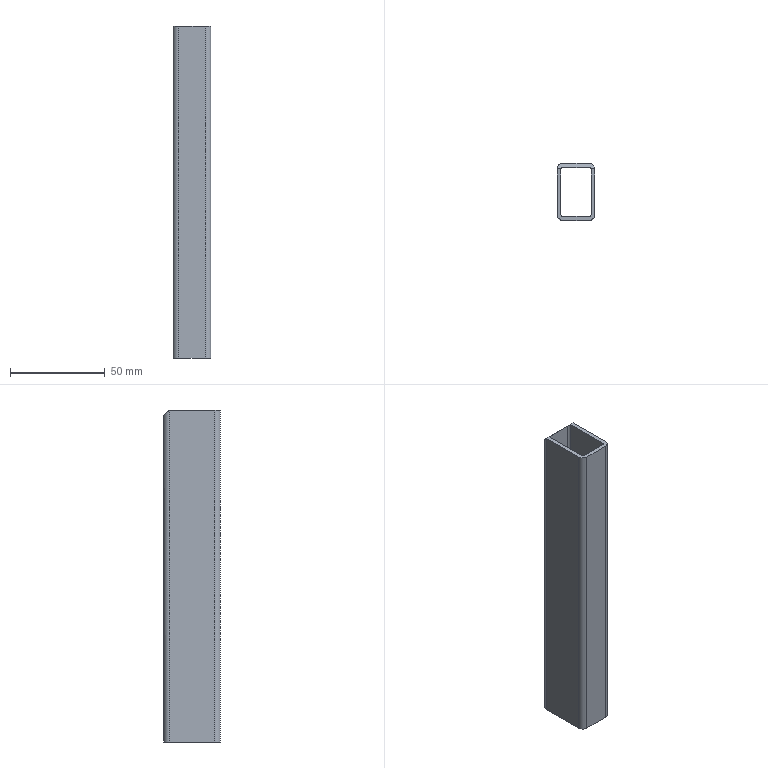Component | SolidWorks | A30x20x2RectangularColdBentHollowSectionSteel175mm-1 | 1 solid | 19 faces | box 20 x 30 x 175 mm | volume 30925 mm3 | plane 11 | cylinder 8 | commonest cylinder face diameters 6 x4 2 x4
build123d program:
from build123d import *

# Parameters (mm, degrees)
BOSS_EXTRUDE1_DEPTH     = 175
CUT_EXTRUDE1_DEPTH      = 176.926
CUT_EXTRUDE1_DEPTH_BACK = 176.926


with BuildPart() as part:
    # Sketch1_2 → Boss-Extrude1 (new body)
    with BuildSketch(Plane(origin=(0, 0, 0), x_dir=(0, 0, -1), z_dir=(1, 0, 0))):
        with BuildLine():
            Line((-6.263, 13), (6.263, 13))
            Line((6.263, 13), (7.561, 14.947))
            ThreePointArc((7.561, 14.947), (7.282, 14.987), (7, 15))
            Line((7, 15), (-7, 15))
            ThreePointArc((-7, 15), (-7.282, 14.987), (-7.561, 14.947))
            Line((-7.561, 14.947), (-6.263, 13))
        make_face()
        with BuildLine():
            Line((-10, -11.394), (-8, -8.394))
            Line((-8, -8.394), (-8, 12))
            ThreePointArc((-8, 12), (-7.707, 12.707), (-7, 13))
            Line((-7, 13), (-6.263, 13))
            Line((-6.263, 13), (-7.561, 14.947))
            ThreePointArc((-7.561, 14.947), (-9.311, 13.913), (-10, 12))
            Line((-10, 12), (-10, -11.394))
        make_face()
        with BuildLine():
            Line((8, 12), (8, -8.394))
            Line((8, -8.394), (10, -11.394))
            Line((10, -11.394), (10, 12))
            ThreePointArc((10, 12), (9.311, 13.913), (7.561, 14.947))
            Line((7.561, 14.947), (6.263, 13))
            Line((6.263, 13), (7, 13))
            ThreePointArc((7, 13), (7.707, 12.707), (8, 12))
        make_face()
        with BuildLine():
            Line((7, -13), (-7, -13))
            ThreePointArc((-7, -13), (-7.707, -12.707), (-8, -12))
            Line((-8, -12), (-8, -8.394))
            Line((-8, -8.394), (-10, -11.394))
            Line((-10, -11.394), (-10, -12))
            ThreePointArc((-10, -12), (-9.121, -14.121), (-7, -15))
            Line((-7, -15), (7, -15))
            ThreePointArc((7, -15), (9.121, -14.121), (10, -12))
            Line((10, -12), (10, -11.394))
            Line((10, -11.394), (8, -8.394))
            Line((8, -8.394), (8, -12))
            ThreePointArc((8, -12), (7.707, -12.707), (7, -13))
        make_face()
    extrude(amount=BOSS_EXTRUDE1_DEPTH)

    # Sketch1 → Cut-Extrude1 (cut, two sides: drawn at the far end of the back side and taken through both)
    with BuildSketch(Plane.XY.offset(-CUT_EXTRUDE1_DEPTH_BACK)):
        Polygon((-1, 11), (-1, 16), (4, 16), align=None)
    extrude(amount=CUT_EXTRUDE1_DEPTH + CUT_EXTRUDE1_DEPTH_BACK, mode=Mode.SUBTRACT)


solid = part.part

# Placed as in the assembly
solid = solid.moved(Location((76.629, 35.1, 413), (0, 90, 0)))
STEP:
#1=COLOUR_RGB('',0.7922,0.8196,0.9333);
#2=FILL_AREA_STYLE_COLOUR('',#1);
#3=FILL_AREA_STYLE('',(#2));
#4=SURFACE_STYLE_FILL_AREA(#3);
#5=SURFACE_SIDE_STYLE('',(#4));
#6=SURFACE_STYLE_USAGE(.BOTH.,#5);
#7=PRESENTATION_STYLE_ASSIGNMENT((#6));
#8=CARTESIAN_POINT('',(3.411,1.854,16.26));
#9=VERTEX_POINT('',#8);
#10=CARTESIAN_POINT('',(3.292,1.972,16.142));
#11=VERTEX_POINT('',#10);
#12=CARTESIAN_POINT('',(3.411,1.854,16.26));
#13=CARTESIAN_POINT('',(3.411,1.924,16.191));
#14=CARTESIAN_POINT('',(3.362,1.972,16.142));
#15=CARTESIAN_POINT('',(3.292,1.972,16.142));
#16=(BOUNDED_CURVE()B_SPLINE_CURVE(3,(#12,#13,#14,#15),.UNSPECIFIED.,.F.,.T.)B_SPLINE_CURVE_WITH_KNOTS((4,4),(1.571,3.142),.UNSPECIFIED.)CURVE()GEOMETRIC_REPRESENTATION_ITEM()RATIONAL_B_SPLINE_CURVE((1.,0.8047,0.8047,1.))REPRESENTATION_ITEM(''));
#17=EDGE_CURVE('',#9,#11,#16,.T.);
#18=ORIENTED_EDGE('',*,*,#17,.F.);
#19=CARTESIAN_POINT('',(3.411,1.854,9.37));
#20=VERTEX_POINT('',#19);
#21=CARTESIAN_POINT('',(3.411,1.854,9.37));
#22=DIRECTION('',(-0.,-0.,1.));
#23=VECTOR('',#22,39.37);
#24=LINE('',#21,#23);
#25=EDGE_CURVE('',#20,#9,#24,.T.);
#26=ORIENTED_EDGE('',*,*,#25,.F.);
#27=CARTESIAN_POINT('',(3.292,1.972,9.37));
#28=VERTEX_POINT('',#27);
#29=CARTESIAN_POINT('',(3.292,1.854,9.37));
#30=DIRECTION('',(-0.,-0.,1.));
#31=DIRECTION('',(-1.,0.,0.));
#32=AXIS2_PLACEMENT_3D('',#29,#30,#31);
#33=CIRCLE('',#32,0.1181);
#34=EDGE_CURVE('',#20,#28,#33,.T.);
#35=ORIENTED_EDGE('',*,*,#34,.T.);
#36=CARTESIAN_POINT('',(3.292,1.972,9.37));
#37=DIRECTION('',(-0.,-0.,1.));
#38=VECTOR('',#37,39.37);
#39=LINE('',#36,#38);
#40=EDGE_CURVE('',#28,#11,#39,.T.);
#41=ORIENTED_EDGE('',*,*,#40,.T.);
#42=EDGE_LOOP('',(#18,#26,#35,#41));
#43=FACE_OUTER_BOUND('',#42,.T.);
#44=CARTESIAN_POINT('',(3.292,1.854,9.37));
#45=DIRECTION('',(-0.,-0.,1.));
#46=DIRECTION('',(1.,0.,0.));
#47=AXIS2_PLACEMENT_3D('',#44,#45,#46);
#48=CYLINDRICAL_SURFACE('',#47,0.1181);
#49=ADVANCED_FACE('',(#43),#48,.T.);
#50=CARTESIAN_POINT('',(3.411,0.9094,16.26));
#51=VERTEX_POINT('',#50);
#52=CARTESIAN_POINT('',(3.411,1.382,16.26));
#53=DIRECTION('',(0.,1.,0.));
#54=VECTOR('',#53,39.37);
#55=LINE('',#52,#54);
#56=EDGE_CURVE('',#51,#9,#55,.T.);
#57=ORIENTED_EDGE('',*,*,#56,.F.);
#58=CARTESIAN_POINT('',(3.411,0.9094,9.37));
#59=VERTEX_POINT('',#58);
#60=CARTESIAN_POINT('',(3.411,0.9094,9.37));
#61=DIRECTION('',(-0.,-0.,1.));
#62=VECTOR('',#61,39.37);
#63=LINE('',#60,#62);
#64=EDGE_CURVE('',#59,#51,#63,.T.);
#65=ORIENTED_EDGE('',*,*,#64,.F.);
#66=CARTESIAN_POINT('',(3.411,1.382,9.37));
#67=DIRECTION('',(0.,1.,0.));
#68=VECTOR('',#67,39.37);
#69=LINE('',#66,#68);
#70=EDGE_CURVE('',#59,#20,#69,.T.);
#71=ORIENTED_EDGE('',*,*,#70,.T.);
#72=ORIENTED_EDGE('',*,*,#25,.T.);
#73=EDGE_LOOP('',(#57,#65,#71,#72));
#74=FACE_OUTER_BOUND('',#73,.T.);
#75=CARTESIAN_POINT('',(3.411,1.382,9.37));
#76=DIRECTION('',(1.,-0.,0.));
#77=DIRECTION('',(0.,0.,-1.));
#78=AXIS2_PLACEMENT_3D('',#75,#76,#77);
#79=PLANE('',#78);
#80=ADVANCED_FACE('',(#74),#79,.T.);
#81=CARTESIAN_POINT('',(3.292,0.7913,16.26));
#82=VERTEX_POINT('',#81);
#83=CARTESIAN_POINT('',(3.292,0.9094,16.26));
#84=DIRECTION('',(-0.,-0.,1.));
#85=DIRECTION('',(-1.,0.,0.));
#86=AXIS2_PLACEMENT_3D('',#83,#84,#85);
#87=CIRCLE('',#86,0.1181);
#88=EDGE_CURVE('',#82,#51,#87,.T.);
#89=ORIENTED_EDGE('',*,*,#88,.F.);
#90=CARTESIAN_POINT('',(3.292,0.7913,9.37));
#91=VERTEX_POINT('',#90);
#92=CARTESIAN_POINT('',(3.292,0.7913,9.37));
#93=DIRECTION('',(-0.,-0.,1.));
#94=VECTOR('',#93,39.37);
#95=LINE('',#92,#94);
#96=EDGE_CURVE('',#91,#82,#95,.T.);
#97=ORIENTED_EDGE('',*,*,#96,.F.);
#98=CARTESIAN_POINT('',(3.292,0.9094,9.37));
#99=DIRECTION('',(-0.,-0.,1.));
#100=DIRECTION('',(-1.,0.,0.));
#101=AXIS2_PLACEMENT_3D('',#98,#99,#100);
#102=CIRCLE('',#101,0.1181);
#103=EDGE_CURVE('',#91,#59,#102,.T.);
#104=ORIENTED_EDGE('',*,*,#103,.T.);
#105=ORIENTED_EDGE('',*,*,#64,.T.);
#106=EDGE_LOOP('',(#89,#97,#104,#105));
#107=FACE_OUTER_BOUND('',#106,.T.);
#108=CARTESIAN_POINT('',(3.292,0.9094,9.37));
#109=DIRECTION('',(-0.,-0.,1.));
#110=DIRECTION('',(1.,0.,0.));
#111=AXIS2_PLACEMENT_3D('',#108,#109,#110);
#112=CYLINDRICAL_SURFACE('',#111,0.1181);
#113=ADVANCED_FACE('',(#107),#112,.T.);
#114=CARTESIAN_POINT('',(2.741,0.7913,16.26));
#115=VERTEX_POINT('',#114);
#116=CARTESIAN_POINT('',(3.017,0.7913,16.26));
#117=DIRECTION('',(-1.,0.,-0.));
#118=VECTOR('',#117,39.37);
#119=LINE('',#116,#118);
#120=EDGE_CURVE('',#82,#115,#119,.T.);
#121=ORIENTED_EDGE('',*,*,#120,.T.);
#122=CARTESIAN_POINT('',(2.741,0.7913,9.37));
#123=VERTEX_POINT('',#122);
#124=CARTESIAN_POINT('',(2.741,0.7913,9.37));
#125=DIRECTION('',(-0.,-0.,1.));
#126=VECTOR('',#125,39.37);
#127=LINE('',#124,#126);
#128=EDGE_CURVE('',#123,#115,#127,.T.);
#129=ORIENTED_EDGE('',*,*,#128,.F.);
#130=CARTESIAN_POINT('',(3.017,0.7913,9.37));
#131=DIRECTION('',(-1.,0.,-0.));
#132=VECTOR('',#131,39.37);
#133=LINE('',#130,#132);
#134=EDGE_CURVE('',#91,#123,#133,.T.);
#135=ORIENTED_EDGE('',*,*,#134,.F.);
#136=ORIENTED_EDGE('',*,*,#96,.T.);
#137=EDGE_LOOP('',(#121,#129,#135,#136));
#138=FACE_OUTER_BOUND('',#137,.T.);
#139=CARTESIAN_POINT('',(3.017,0.7913,9.37));
#140=DIRECTION('',(0.,1.,0.));
#141=DIRECTION('',(1.,-0.,0.));
#142=AXIS2_PLACEMENT_3D('',#139,#140,#141);
#143=PLANE('',#142);
#144=ADVANCED_FACE('',(#138),#143,.F.);
#145=CARTESIAN_POINT('',(2.623,0.9094,16.26));
#146=VERTEX_POINT('',#145);
#147=CARTESIAN_POINT('',(2.741,0.9094,16.26));
#148=DIRECTION('',(0.,0.,-1.));
#149=DIRECTION('',(-1.,0.,0.));
#150=AXIS2_PLACEMENT_3D('',#147,#148,#149);
#151=CIRCLE('',#150,0.1181);
#152=EDGE_CURVE('',#115,#146,#151,.T.);
#153=ORIENTED_EDGE('',*,*,#152,.T.);
#154=CARTESIAN_POINT('',(2.623,0.9094,9.37));
#155=VERTEX_POINT('',#154);
#156=CARTESIAN_POINT('',(2.623,0.9094,9.37));
#157=DIRECTION('',(-0.,-0.,1.));
#158=VECTOR('',#157,39.37);
#159=LINE('',#156,#158);
#160=EDGE_CURVE('',#155,#146,#159,.T.);
#161=ORIENTED_EDGE('',*,*,#160,.F.);
#162=CARTESIAN_POINT('',(2.741,0.9094,9.37));
#163=DIRECTION('',(0.,0.,-1.));
#164=DIRECTION('',(-1.,0.,0.));
#165=AXIS2_PLACEMENT_3D('',#162,#163,#164);
#166=CIRCLE('',#165,0.1181);
#167=EDGE_CURVE('',#123,#155,#166,.T.);
#168=ORIENTED_EDGE('',*,*,#167,.F.);
#169=ORIENTED_EDGE('',*,*,#128,.T.);
#170=EDGE_LOOP('',(#153,#161,#168,#169));
#171=FACE_OUTER_BOUND('',#170,.T.);
#172=CARTESIAN_POINT('',(2.741,0.9094,9.37));
#173=DIRECTION('',(-0.,-0.,1.));
#174=DIRECTION('',(1.,0.,0.));
#175=AXIS2_PLACEMENT_3D('',#172,#173,#174);
#176=CYLINDRICAL_SURFACE('',#175,0.1181);
#177=ADVANCED_FACE('',(#171),#176,.T.);
#178=CARTESIAN_POINT('',(2.623,1.854,16.26));
#179=VERTEX_POINT('',#178);
#180=CARTESIAN_POINT('',(2.623,1.382,16.26));
#181=DIRECTION('',(0.,1.,0.));
#182=VECTOR('',#181,39.37);
#183=LINE('',#180,#182);
#184=EDGE_CURVE('',#146,#179,#183,.T.);
#185=ORIENTED_EDGE('',*,*,#184,.T.);
#186=CARTESIAN_POINT('',(2.623,1.854,9.37));
#187=VERTEX_POINT('',#186);
#188=CARTESIAN_POINT('',(2.623,1.854,9.37));
#189=DIRECTION('',(-0.,-0.,1.));
#190=VECTOR('',#189,39.37);
#191=LINE('',#188,#190);
#192=EDGE_CURVE('',#187,#179,#191,.T.);
#193=ORIENTED_EDGE('',*,*,#192,.F.);
#194=CARTESIAN_POINT('',(2.623,1.382,9.37));
#195=DIRECTION('',(0.,1.,0.));
#196=VECTOR('',#195,39.37);
#197=LINE('',#194,#196);
#198=EDGE_CURVE('',#155,#187,#197,.T.);
#199=ORIENTED_EDGE('',*,*,#198,.F.);
#200=ORIENTED_EDGE('',*,*,#160,.T.);
#201=EDGE_LOOP('',(#185,#193,#199,#200));
#202=FACE_OUTER_BOUND('',#201,.T.);
#203=CARTESIAN_POINT('',(2.623,1.382,9.37));
#204=DIRECTION('',(1.,-0.,0.));
#205=DIRECTION('',(0.,0.,-1.));
#206=AXIS2_PLACEMENT_3D('',#203,#204,#205);
#207=PLANE('',#206);
#208=ADVANCED_FACE('',(#202),#207,.F.);
#209=CARTESIAN_POINT('',(2.741,1.972,16.142));
#210=VERTEX_POINT('',#209);
#211=CARTESIAN_POINT('',(2.741,1.972,16.142));
#212=CARTESIAN_POINT('',(2.672,1.972,16.142));
#213=CARTESIAN_POINT('',(2.623,1.924,16.191));
#214=CARTESIAN_POINT('',(2.623,1.854,16.26));
#215=(BOUNDED_CURVE()B_SPLINE_CURVE(3,(#211,#212,#213,#214),.UNSPECIFIED.,.F.,.T.)B_SPLINE_CURVE_WITH_KNOTS((4,4),(3.142,4.712),.UNSPECIFIED.)CURVE()GEOMETRIC_REPRESENTATION_ITEM()RATIONAL_B_SPLINE_CURVE((1.,0.8047,0.8047,1.))REPRESENTATION_ITEM(''));
#216=EDGE_CURVE('',#210,#179,#215,.T.);
#217=ORIENTED_EDGE('',*,*,#216,.F.);
#218=CARTESIAN_POINT('',(2.741,1.972,9.37));
#219=VERTEX_POINT('',#218);
#220=CARTESIAN_POINT('',(2.741,1.972,9.37));
#221=DIRECTION('',(-0.,-0.,1.));
#222=VECTOR('',#221,39.37);
#223=LINE('',#220,#222);
#224=EDGE_CURVE('',#219,#210,#223,.T.);
#225=ORIENTED_EDGE('',*,*,#224,.F.);
#226=CARTESIAN_POINT('',(2.741,1.854,9.37));
#227=DIRECTION('',(-0.,-0.,1.));
#228=DIRECTION('',(-1.,0.,0.));
#229=AXIS2_PLACEMENT_3D('',#226,#227,#228);
#230=CIRCLE('',#229,0.1181);
#231=EDGE_CURVE('',#219,#187,#230,.T.);
#232=ORIENTED_EDGE('',*,*,#231,.T.);
#233=ORIENTED_EDGE('',*,*,#192,.T.);
#234=EDGE_LOOP('',(#217,#225,#232,#233));
#235=FACE_OUTER_BOUND('',#234,.T.);
#236=CARTESIAN_POINT('',(2.741,1.854,9.37));
#237=DIRECTION('',(-0.,-0.,1.));
#238=DIRECTION('',(1.,0.,0.));
#239=AXIS2_PLACEMENT_3D('',#236,#237,#238);
#240=CYLINDRICAL_SURFACE('',#239,0.1181);
#241=ADVANCED_FACE('',(#235),#240,.T.);
#242=CARTESIAN_POINT('',(3.292,0.8701,16.26));
#243=VERTEX_POINT('',#242);
#244=CARTESIAN_POINT('',(3.332,0.9094,16.26));
#245=VERTEX_POINT('',#244);
#246=CARTESIAN_POINT('',(3.292,0.9094,16.26));
#247=DIRECTION('',(-0.,-0.,1.));
#248=DIRECTION('',(-1.,0.,0.));
#249=AXIS2_PLACEMENT_3D('',#246,#247,#248);
#250=CIRCLE('',#249,0.03937);
#251=EDGE_CURVE('',#243,#245,#250,.T.);
#252=ORIENTED_EDGE('',*,*,#251,.T.);
#253=CARTESIAN_POINT('',(3.332,0.9094,9.37));
#254=VERTEX_POINT('',#253);
#255=CARTESIAN_POINT('',(3.332,0.9094,9.37));
#256=DIRECTION('',(-0.,-0.,1.));
#257=VECTOR('',#256,39.37);
#258=LINE('',#255,#257);
#259=EDGE_CURVE('',#254,#245,#258,.T.);
#260=ORIENTED_EDGE('',*,*,#259,.F.);
#261=CARTESIAN_POINT('',(3.292,0.8701,9.37));
#262=VERTEX_POINT('',#261);
#263=CARTESIAN_POINT('',(3.292,0.9094,9.37));
#264=DIRECTION('',(-0.,-0.,1.));
#265=DIRECTION('',(-1.,0.,0.));
#266=AXIS2_PLACEMENT_3D('',#263,#264,#265);
#267=CIRCLE('',#266,0.03937);
#268=EDGE_CURVE('',#262,#254,#267,.T.);
#269=ORIENTED_EDGE('',*,*,#268,.F.);
#270=CARTESIAN_POINT('',(3.292,0.8701,9.37));
#271=DIRECTION('',(-0.,-0.,1.));
#272=VECTOR('',#271,39.37);
#273=LINE('',#270,#272);
#274=EDGE_CURVE('',#262,#243,#273,.T.);
#275=ORIENTED_EDGE('',*,*,#274,.T.);
#276=EDGE_LOOP('',(#252,#260,#269,#275));
#277=FACE_OUTER_BOUND('',#276,.T.);
#278=CARTESIAN_POINT('',(3.292,0.9094,9.37));
#279=DIRECTION('',(-0.,-0.,1.));
#280=DIRECTION('',(1.,0.,0.));
#281=AXIS2_PLACEMENT_3D('',#278,#279,#280);
#282=CYLINDRICAL_SURFACE('',#281,0.03937);
#283=ADVANCED_FACE('',(#277),#282,.F.);
#284=CARTESIAN_POINT('',(3.332,1.854,16.26));
#285=VERTEX_POINT('',#284);
#286=CARTESIAN_POINT('',(3.332,1.382,16.26));
#287=DIRECTION('',(0.,1.,0.));
#288=VECTOR('',#287,39.37);
#289=LINE('',#286,#288);
#290=EDGE_CURVE('',#245,#285,#289,.T.);
#291=ORIENTED_EDGE('',*,*,#290,.T.);
#292=CARTESIAN_POINT('',(3.332,1.854,9.37));
#293=VERTEX_POINT('',#292);
#294=CARTESIAN_POINT('',(3.332,1.854,9.37));
#295=DIRECTION('',(-0.,-0.,1.));
#296=VECTOR('',#295,39.37);
#297=LINE('',#294,#296);
#298=EDGE_CURVE('',#293,#285,#297,.T.);
#299=ORIENTED_EDGE('',*,*,#298,.F.);
#300=CARTESIAN_POINT('',(3.332,1.382,9.37));
#301=DIRECTION('',(0.,1.,0.));
#302=VECTOR('',#301,39.37);
#303=LINE('',#300,#302);
#304=EDGE_CURVE('',#254,#293,#303,.T.);
#305=ORIENTED_EDGE('',*,*,#304,.F.);
#306=ORIENTED_EDGE('',*,*,#259,.T.);
#307=EDGE_LOOP('',(#291,#299,#305,#306));
#308=FACE_OUTER_BOUND('',#307,.T.);
#309=CARTESIAN_POINT('',(3.332,1.382,9.37));
#310=DIRECTION('',(1.,-0.,0.));
#311=DIRECTION('',(0.,0.,-1.));
#312=AXIS2_PLACEMENT_3D('',#309,#310,#311);
#313=PLANE('',#312);
#314=ADVANCED_FACE('',(#308),#313,.F.);
#315=ORIENTED_EDGE('',*,*,#298,.T.);
#316=CARTESIAN_POINT('',(3.292,1.894,16.22));
#317=VERTEX_POINT('',#316);
#318=CARTESIAN_POINT('',(3.332,1.854,16.26));
#319=CARTESIAN_POINT('',(3.332,1.877,16.237));
#320=CARTESIAN_POINT('',(3.316,1.894,16.22));
#321=CARTESIAN_POINT('',(3.292,1.894,16.22));
#322=(BOUNDED_CURVE()B_SPLINE_CURVE(3,(#318,#319,#320,#321),.UNSPECIFIED.,.F.,.T.)B_SPLINE_CURVE_WITH_KNOTS((4,4),(1.571,3.142),.UNSPECIFIED.)CURVE()GEOMETRIC_REPRESENTATION_ITEM()RATIONAL_B_SPLINE_CURVE((1.,0.8047,0.8047,1.))REPRESENTATION_ITEM(''));
#323=EDGE_CURVE('',#285,#317,#322,.T.);
#324=ORIENTED_EDGE('',*,*,#323,.T.);
#325=CARTESIAN_POINT('',(3.292,1.894,9.37));
#326=VERTEX_POINT('',#325);
#327=CARTESIAN_POINT('',(3.292,1.894,9.37));
#328=DIRECTION('',(-0.,-0.,1.));
#329=VECTOR('',#328,39.37);
#330=LINE('',#327,#329);
#331=EDGE_CURVE('',#326,#317,#330,.T.);
#332=ORIENTED_EDGE('',*,*,#331,.F.);
#333=CARTESIAN_POINT('',(3.292,1.854,9.37));
#334=DIRECTION('',(-0.,-0.,1.));
#335=DIRECTION('',(-1.,0.,0.));
#336=AXIS2_PLACEMENT_3D('',#333,#334,#335);
#337=CIRCLE('',#336,0.03937);
#338=EDGE_CURVE('',#293,#326,#337,.T.);
#339=ORIENTED_EDGE('',*,*,#338,.F.);
#340=EDGE_LOOP('',(#315,#324,#332,#339));
#341=FACE_OUTER_BOUND('',#340,.T.);
#342=CARTESIAN_POINT('',(3.292,1.854,9.37));
#343=DIRECTION('',(-0.,-0.,1.));
#344=DIRECTION('',(1.,0.,0.));
#345=AXIS2_PLACEMENT_3D('',#342,#343,#344);
#346=CYLINDRICAL_SURFACE('',#345,0.03937);
#347=ADVANCED_FACE('',(#341),#346,.F.);
#348=ORIENTED_EDGE('',*,*,#331,.T.);
#349=CARTESIAN_POINT('',(2.741,1.894,16.22));
#350=VERTEX_POINT('',#349);
#351=CARTESIAN_POINT('',(3.017,1.894,16.22));
#352=DIRECTION('',(-1.,0.,-0.));
#353=VECTOR('',#352,39.37);
#354=LINE('',#351,#353);
#355=EDGE_CURVE('',#317,#350,#354,.T.);
#356=ORIENTED_EDGE('',*,*,#355,.T.);
#357=CARTESIAN_POINT('',(2.741,1.894,9.37));
#358=VERTEX_POINT('',#357);
#359=CARTESIAN_POINT('',(2.741,1.894,9.37));
#360=DIRECTION('',(-0.,-0.,1.));
#361=VECTOR('',#360,39.37);
#362=LINE('',#359,#361);
#363=EDGE_CURVE('',#358,#350,#362,.T.);
#364=ORIENTED_EDGE('',*,*,#363,.F.);
#365=CARTESIAN_POINT('',(3.017,1.894,9.37));
#366=DIRECTION('',(-1.,0.,-0.));
#367=VECTOR('',#366,39.37);
#368=LINE('',#365,#367);
#369=EDGE_CURVE('',#326,#358,#368,.T.);
#370=ORIENTED_EDGE('',*,*,#369,.F.);
#371=EDGE_LOOP('',(#348,#356,#364,#370));
#372=FACE_OUTER_BOUND('',#371,.T.);
#373=CARTESIAN_POINT('',(3.017,1.894,9.37));
#374=DIRECTION('',(0.,1.,0.));
#375=DIRECTION('',(1.,-0.,0.));
#376=AXIS2_PLACEMENT_3D('',#373,#374,#375);
#377=PLANE('',#376);
#378=ADVANCED_FACE('',(#372),#377,.F.);
#379=ORIENTED_EDGE('',*,*,#363,.T.);
#380=CARTESIAN_POINT('',(2.702,1.854,16.26));
#381=VERTEX_POINT('',#380);
#382=CARTESIAN_POINT('',(2.741,1.894,16.22));
#383=CARTESIAN_POINT('',(2.718,1.894,16.22));
#384=CARTESIAN_POINT('',(2.702,1.877,16.237));
#385=CARTESIAN_POINT('',(2.702,1.854,16.26));
#386=(BOUNDED_CURVE()B_SPLINE_CURVE(3,(#382,#383,#384,#385),.UNSPECIFIED.,.F.,.T.)B_SPLINE_CURVE_WITH_KNOTS((4,4),(3.142,4.712),.UNSPECIFIED.)CURVE()GEOMETRIC_REPRESENTATION_ITEM()RATIONAL_B_SPLINE_CURVE((1.,0.8047,0.8047,1.))REPRESENTATION_ITEM(''));
#387=EDGE_CURVE('',#350,#381,#386,.T.);
#388=ORIENTED_EDGE('',*,*,#387,.T.);
#389=CARTESIAN_POINT('',(2.702,1.854,9.37));
#390=VERTEX_POINT('',#389);
#391=CARTESIAN_POINT('',(2.702,1.854,9.37));
#392=DIRECTION('',(-0.,-0.,1.));
#393=VECTOR('',#392,39.37);
#394=LINE('',#391,#393);
#395=EDGE_CURVE('',#390,#381,#394,.T.);
#396=ORIENTED_EDGE('',*,*,#395,.F.);
#397=CARTESIAN_POINT('',(2.741,1.854,9.37));
#398=DIRECTION('',(-0.,-0.,1.));
#399=DIRECTION('',(-1.,0.,0.));
#400=AXIS2_PLACEMENT_3D('',#397,#398,#399);
#401=CIRCLE('',#400,0.03937);
#402=EDGE_CURVE('',#358,#390,#401,.T.);
#403=ORIENTED_EDGE('',*,*,#402,.F.);
#404=EDGE_LOOP('',(#379,#388,#396,#403));
#405=FACE_OUTER_BOUND('',#404,.T.);
#406=CARTESIAN_POINT('',(2.741,1.854,9.37));
#407=DIRECTION('',(-0.,-0.,1.));
#408=DIRECTION('',(1.,0.,0.));
#409=AXIS2_PLACEMENT_3D('',#406,#407,#408);
#410=CYLINDRICAL_SURFACE('',#409,0.03937);
#411=ADVANCED_FACE('',(#405),#410,.F.);
#412=CARTESIAN_POINT('',(2.702,0.9094,16.26));
#413=VERTEX_POINT('',#412);
#414=CARTESIAN_POINT('',(2.702,1.382,16.26));
#415=DIRECTION('',(0.,1.,0.));
#416=VECTOR('',#415,39.37);
#417=LINE('',#414,#416);
#418=EDGE_CURVE('',#413,#381,#417,.T.);
#419=ORIENTED_EDGE('',*,*,#418,.F.);
#420=CARTESIAN_POINT('',(2.702,0.9094,9.37));
#421=VERTEX_POINT('',#420);
#422=CARTESIAN_POINT('',(2.702,0.9094,9.37));
#423=DIRECTION('',(-0.,-0.,1.));
#424=VECTOR('',#423,39.37);
#425=LINE('',#422,#424);
#426=EDGE_CURVE('',#421,#413,#425,.T.);
#427=ORIENTED_EDGE('',*,*,#426,.F.);
#428=CARTESIAN_POINT('',(2.702,1.382,9.37));
#429=DIRECTION('',(0.,1.,0.));
#430=VECTOR('',#429,39.37);
#431=LINE('',#428,#430);
#432=EDGE_CURVE('',#421,#390,#431,.T.);
#433=ORIENTED_EDGE('',*,*,#432,.T.);
#434=ORIENTED_EDGE('',*,*,#395,.T.);
#435=EDGE_LOOP('',(#419,#427,#433,#434));
#436=FACE_OUTER_BOUND('',#435,.T.);
#437=CARTESIAN_POINT('',(2.702,1.382,9.37));
#438=DIRECTION('',(1.,-0.,0.));
#439=DIRECTION('',(0.,0.,-1.));
#440=AXIS2_PLACEMENT_3D('',#437,#438,#439);
#441=PLANE('',#440);
#442=ADVANCED_FACE('',(#436),#441,.T.);
#443=CARTESIAN_POINT('',(2.741,0.8701,16.26));
#444=VERTEX_POINT('',#443);
#445=CARTESIAN_POINT('',(2.741,0.9094,16.26));
#446=DIRECTION('',(0.,0.,-1.));
#447=DIRECTION('',(-1.,0.,0.));
#448=AXIS2_PLACEMENT_3D('',#445,#446,#447);
#449=CIRCLE('',#448,0.03937);
#450=EDGE_CURVE('',#444,#413,#449,.T.);
#451=ORIENTED_EDGE('',*,*,#450,.F.);
#452=CARTESIAN_POINT('',(2.741,0.8701,9.37));
#453=VERTEX_POINT('',#452);
#454=CARTESIAN_POINT('',(2.741,0.8701,9.37));
#455=DIRECTION('',(-0.,-0.,1.));
#456=VECTOR('',#455,39.37);
#457=LINE('',#454,#456);
#458=EDGE_CURVE('',#453,#444,#457,.T.);
#459=ORIENTED_EDGE('',*,*,#458,.F.);
#460=CARTESIAN_POINT('',(2.741,0.9094,9.37));
#461=DIRECTION('',(0.,0.,-1.));
#462=DIRECTION('',(-1.,0.,0.));
#463=AXIS2_PLACEMENT_3D('',#460,#461,#462);
#464=CIRCLE('',#463,0.03937);
#465=EDGE_CURVE('',#453,#421,#464,.T.);
#466=ORIENTED_EDGE('',*,*,#465,.T.);
#467=ORIENTED_EDGE('',*,*,#426,.T.);
#468=EDGE_LOOP('',(#451,#459,#466,#467));
#469=FACE_OUTER_BOUND('',#468,.T.);
#470=CARTESIAN_POINT('',(2.741,0.9094,9.37));
#471=DIRECTION('',(-0.,-0.,1.));
#472=DIRECTION('',(1.,0.,0.));
#473=AXIS2_PLACEMENT_3D('',#470,#471,#472);
#474=CYLINDRICAL_SURFACE('',#473,0.03937);
#475=ADVANCED_FACE('',(#469),#474,.F.);
#476=CARTESIAN_POINT('',(3.017,0.8701,16.26));
#477=DIRECTION('',(-1.,0.,-0.));
#478=VECTOR('',#477,39.37);
#479=LINE('',#476,#478);
#480=EDGE_CURVE('',#243,#444,#479,.T.);
#481=ORIENTED_EDGE('',*,*,#480,.F.);
#482=ORIENTED_EDGE('',*,*,#274,.F.);
#483=CARTESIAN_POINT('',(3.017,0.8701,9.37));
#484=DIRECTION('',(-1.,0.,-0.));
#485=VECTOR('',#484,39.37);
#486=LINE('',#483,#485);
#487=EDGE_CURVE('',#262,#453,#486,.T.);
#488=ORIENTED_EDGE('',*,*,#487,.T.);
#489=ORIENTED_EDGE('',*,*,#458,.T.);
#490=EDGE_LOOP('',(#481,#482,#488,#489));
#491=FACE_OUTER_BOUND('',#490,.T.);
#492=CARTESIAN_POINT('',(3.017,0.8701,9.37));
#493=DIRECTION('',(0.,1.,0.));
#494=DIRECTION('',(1.,-0.,0.));
#495=AXIS2_PLACEMENT_3D('',#492,#493,#494);
#496=PLANE('',#495);
#497=ADVANCED_FACE('',(#491),#496,.T.);
#498=CARTESIAN_POINT('',(3.017,1.972,16.142));
#499=DIRECTION('',(-1.,0.,-0.));
#500=VECTOR('',#499,39.37);
#501=LINE('',#498,#500);
#502=EDGE_CURVE('',#11,#210,#501,.T.);
#503=ORIENTED_EDGE('',*,*,#502,.F.);
#504=ORIENTED_EDGE('',*,*,#40,.F.);
#505=CARTESIAN_POINT('',(3.017,1.972,9.37));
#506=DIRECTION('',(-1.,0.,-0.));
#507=VECTOR('',#506,39.37);
#508=LINE('',#505,#507);
#509=EDGE_CURVE('',#28,#219,#508,.T.);
#510=ORIENTED_EDGE('',*,*,#509,.T.);
#511=ORIENTED_EDGE('',*,*,#224,.T.);
#512=EDGE_LOOP('',(#503,#504,#510,#511));
#513=FACE_OUTER_BOUND('',#512,.T.);
#514=CARTESIAN_POINT('',(3.017,1.972,9.37));
#515=DIRECTION('',(0.,1.,0.));
#516=DIRECTION('',(1.,-0.,0.));
#517=AXIS2_PLACEMENT_3D('',#514,#515,#516);
#518=PLANE('',#517);
#519=ADVANCED_FACE('',(#513),#518,.T.);
#520=ORIENTED_EDGE('',*,*,#268,.T.);
#521=ORIENTED_EDGE('',*,*,#304,.T.);
#522=ORIENTED_EDGE('',*,*,#338,.T.);
#523=ORIENTED_EDGE('',*,*,#369,.T.);
#524=ORIENTED_EDGE('',*,*,#402,.T.);
#525=ORIENTED_EDGE('',*,*,#432,.F.);
#526=ORIENTED_EDGE('',*,*,#465,.F.);
#527=ORIENTED_EDGE('',*,*,#487,.F.);
#528=EDGE_LOOP('',(#520,#521,#522,#523,#524,#525,#526,#527));
#529=FACE_BOUND('',#528,.T.);
#530=ORIENTED_EDGE('',*,*,#34,.F.);
#531=ORIENTED_EDGE('',*,*,#70,.F.);
#532=ORIENTED_EDGE('',*,*,#103,.F.);
#533=ORIENTED_EDGE('',*,*,#134,.T.);
#534=ORIENTED_EDGE('',*,*,#167,.T.);
#535=ORIENTED_EDGE('',*,*,#198,.T.);
#536=ORIENTED_EDGE('',*,*,#231,.F.);
#537=ORIENTED_EDGE('',*,*,#509,.F.);
#538=EDGE_LOOP('',(#530,#531,#532,#533,#534,#535,#536,#537));
#539=FACE_OUTER_BOUND('',#538,.T.);
#540=CARTESIAN_POINT('',(3.017,1.382,9.37));
#541=DIRECTION('',(0.,0.,-1.));
#542=DIRECTION('',(-1.,0.,-0.));
#543=AXIS2_PLACEMENT_3D('',#540,#541,#542);
#544=PLANE('',#543);
#545=ADVANCED_FACE('',(#529,#539),#544,.T.);
#546=ORIENTED_EDGE('',*,*,#56,.T.);
#547=CARTESIAN_POINT('',(3.017,1.854,16.26));
#548=DIRECTION('',(-1.,0.,-0.));
#549=VECTOR('',#548,39.37);
#550=LINE('',#547,#549);
#551=EDGE_CURVE('',#9,#285,#550,.T.);
#552=ORIENTED_EDGE('',*,*,#551,.T.);
#553=ORIENTED_EDGE('',*,*,#290,.F.);
#554=ORIENTED_EDGE('',*,*,#251,.F.);
#555=ORIENTED_EDGE('',*,*,#480,.T.);
#556=ORIENTED_EDGE('',*,*,#450,.T.);
#557=ORIENTED_EDGE('',*,*,#418,.T.);
#558=CARTESIAN_POINT('',(3.017,1.854,16.26));
#559=DIRECTION('',(-1.,0.,-0.));
#560=VECTOR('',#559,39.37);
#561=LINE('',#558,#560);
#562=EDGE_CURVE('',#381,#179,#561,.T.);
#563=ORIENTED_EDGE('',*,*,#562,.T.);
#564=ORIENTED_EDGE('',*,*,#184,.F.);
#565=ORIENTED_EDGE('',*,*,#152,.F.);
#566=ORIENTED_EDGE('',*,*,#120,.F.);
#567=ORIENTED_EDGE('',*,*,#88,.T.);
#568=EDGE_LOOP('',(#546,#552,#553,#554,#555,#556,#557,#563,#564,#565,#566,#567));
#569=FACE_OUTER_BOUND('',#568,.T.);
#570=CARTESIAN_POINT('',(3.017,1.382,16.26));
#571=DIRECTION('',(0.,0.,-1.));
#572=DIRECTION('',(-1.,0.,-0.));
#573=AXIS2_PLACEMENT_3D('',#570,#571,#572);
#574=PLANE('',#573);
#575=ADVANCED_FACE('',(#569),#574,.F.);
#576=ORIENTED_EDGE('',*,*,#17,.T.);
#577=ORIENTED_EDGE('',*,*,#502,.T.);
#578=ORIENTED_EDGE('',*,*,#216,.T.);
#579=ORIENTED_EDGE('',*,*,#562,.F.);
#580=ORIENTED_EDGE('',*,*,#387,.F.);
#581=ORIENTED_EDGE('',*,*,#355,.F.);
#582=ORIENTED_EDGE('',*,*,#323,.F.);
#583=ORIENTED_EDGE('',*,*,#551,.F.);
#584=EDGE_LOOP('',(#576,#577,#578,#579,#580,#581,#582,#583));
#585=FACE_OUTER_BOUND('',#584,.T.);
#586=CARTESIAN_POINT('',(2.623,2.012,16.102));
#587=DIRECTION('',(-0.,-0.7071,-0.7071));
#588=DIRECTION('',(0.,0.7071,-0.7071));
#589=AXIS2_PLACEMENT_3D('',#586,#587,#588);
#590=PLANE('',#589);
#591=ADVANCED_FACE('',(#585),#590,.F.);
#592=CLOSED_SHELL('',(#49,#80,#113,#144,#177,#208,#241,#283,#314,#347,#378,#411,#442,#475,#497,#519,#545,#575,#591));
#593=MANIFOLD_SOLID_BREP('',#592);
#594=STYLED_ITEM('',(#7),#593);
#595=(LENGTH_UNIT()NAMED_UNIT(*)SI_UNIT($,.METRE.));
#596=LENGTH_MEASURE_WITH_UNIT(LENGTH_MEASURE(0.0254),#595);
#597=DIMENSIONAL_EXPONENTS(1.,0.,0.,0.,0.,0.,0.);
#598=(CONVERSION_BASED_UNIT('',#596)LENGTH_UNIT()NAMED_UNIT(#597));
#599=UNCERTAINTY_MEASURE_WITH_UNIT(LENGTH_MEASURE(0.00001),#598,'','');
#600=(NAMED_UNIT(*)PLANE_ANGLE_UNIT()SI_UNIT($,.RADIAN.));
#601=(NAMED_UNIT(*)SI_UNIT($,.STERADIAN.)SOLID_ANGLE_UNIT());
#602=(GEOMETRIC_REPRESENTATION_CONTEXT(3)GLOBAL_UNCERTAINTY_ASSIGNED_CONTEXT((#599))GLOBAL_UNIT_ASSIGNED_CONTEXT((#598,#600,#601))REPRESENTATION_CONTEXT('',''));
#603=MECHANICAL_DESIGN_GEOMETRIC_PRESENTATION_REPRESENTATION('',(#594),#602);
#604=CARTESIAN_POINT('',(0.,0.,0.));
#605=DIRECTION('',(0.,0.,1.));
#606=DIRECTION('',(1.,0.,0.));
#607=AXIS2_PLACEMENT_3D('',#604,#605,#606);
#608=(LENGTH_UNIT()NAMED_UNIT(*)SI_UNIT($,.METRE.));
#609=LENGTH_MEASURE_WITH_UNIT(LENGTH_MEASURE(0.0254),#608);
#610=DIMENSIONAL_EXPONENTS(1.,0.,0.,0.,0.,0.,0.);
#611=(CONVERSION_BASED_UNIT('',#609)LENGTH_UNIT()NAMED_UNIT(#610));
#612=UNCERTAINTY_MEASURE_WITH_UNIT(LENGTH_MEASURE(0.00001),#611,'','');
#613=(NAMED_UNIT(*)PLANE_ANGLE_UNIT()SI_UNIT($,.RADIAN.));
#614=(NAMED_UNIT(*)SI_UNIT($,.STERADIAN.)SOLID_ANGLE_UNIT());
#615=(GEOMETRIC_REPRESENTATION_CONTEXT(3)GLOBAL_UNCERTAINTY_ASSIGNED_CONTEXT((#612))GLOBAL_UNIT_ASSIGNED_CONTEXT((#611,#613,#614))REPRESENTATION_CONTEXT('',''));
#616=ADVANCED_BREP_SHAPE_REPRESENTATION('',(#593,#607),#615);
#617=PRESENTATION_LAYER_ASSIGNMENT('','',(#594));